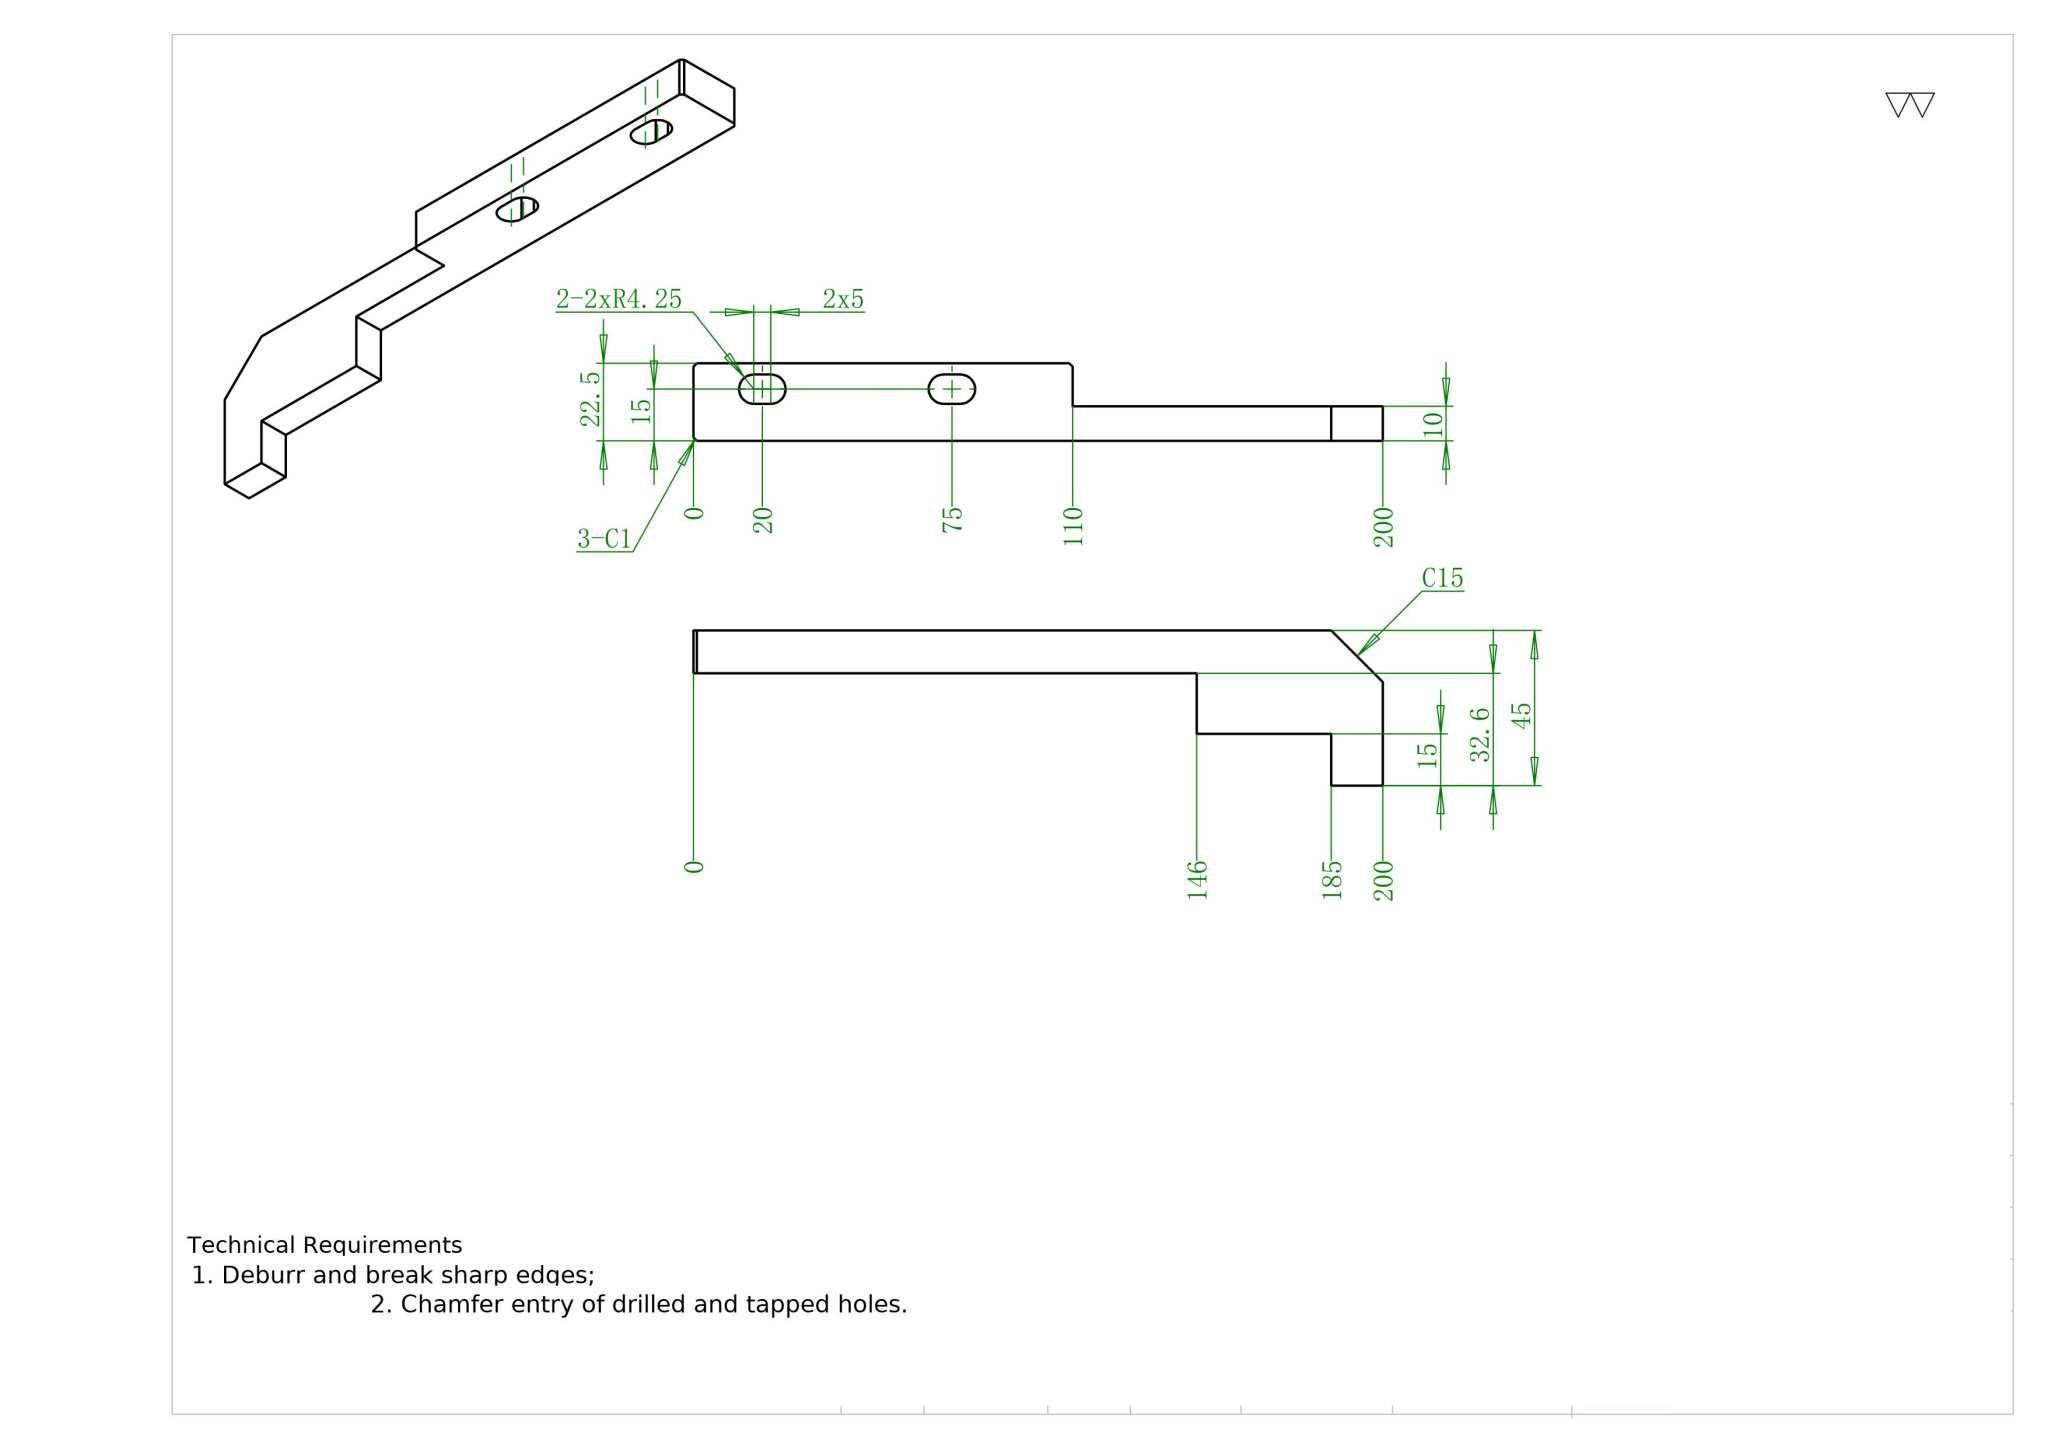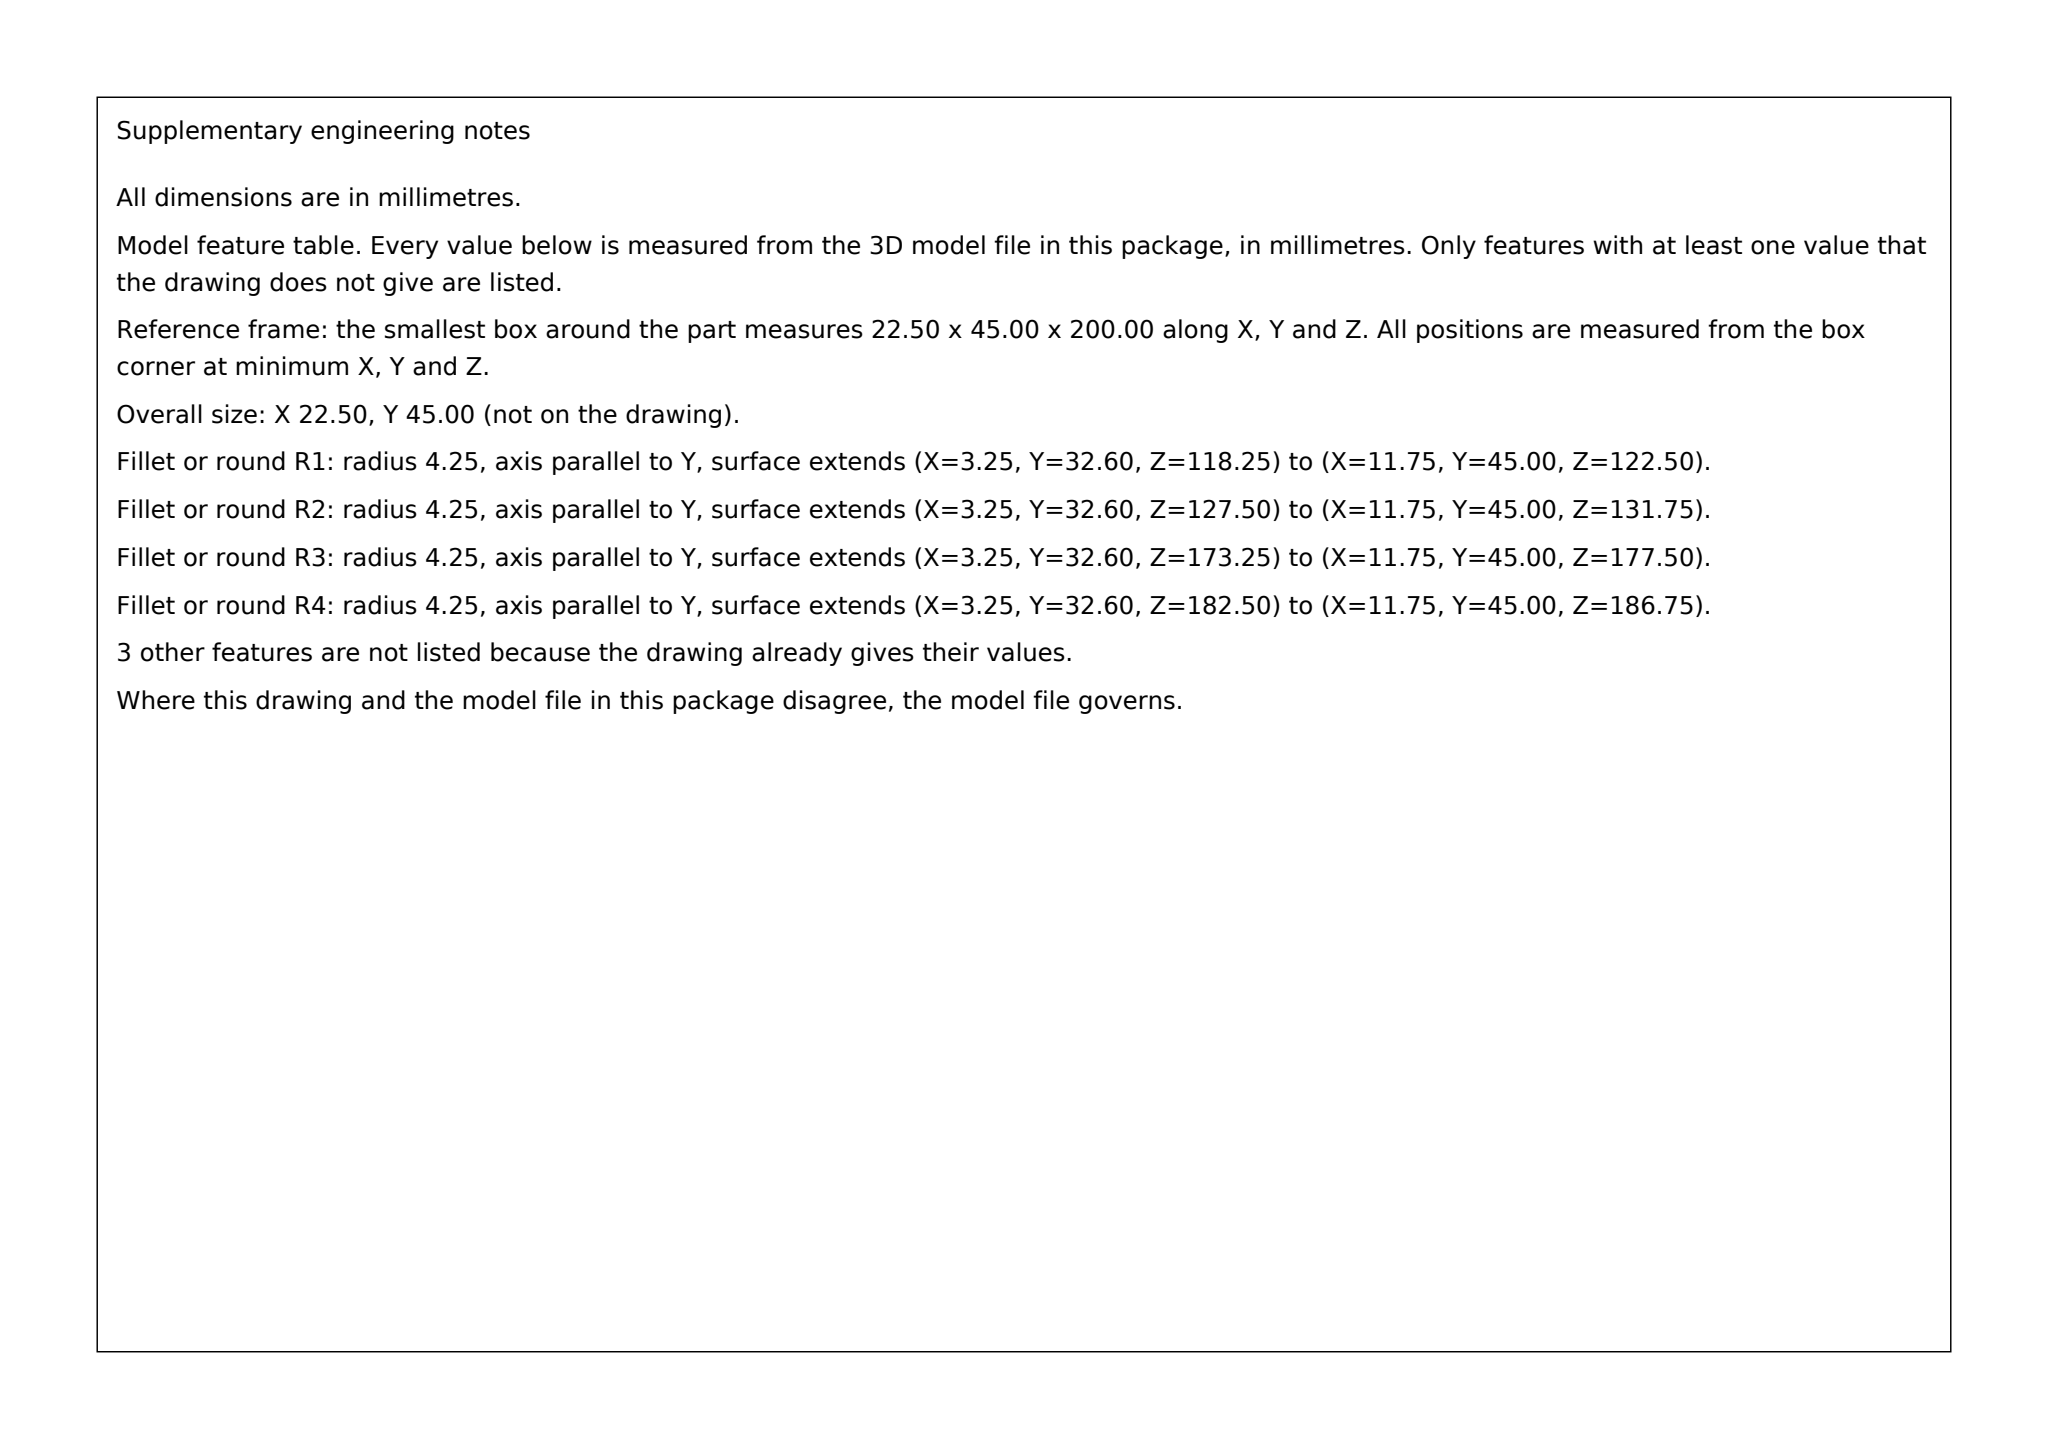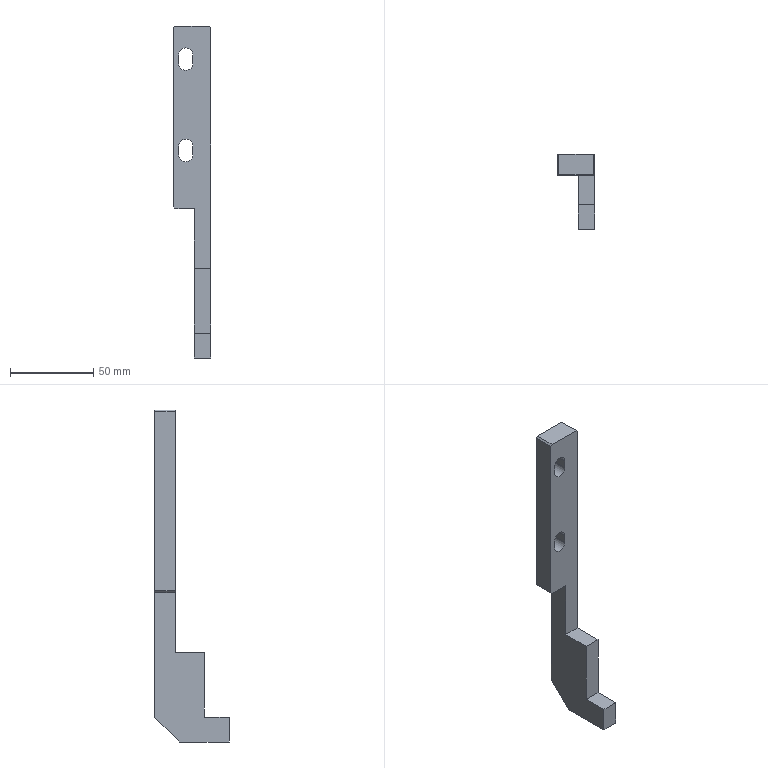Part | SolidWorks | mm | 1 solid | 26 faces | box 22.5 x 45 x 200 mm | volume 49999 mm3 | plane 20 | cylinder 6 | commonest cylinder face diameters 8.5 x6
build123d program:
from build123d import *

# Parameters (mm, degrees)
SKETCH1_W                  = 10
SKETCH1_H                  = 200
BOSS_EXTRUDE1_DEPTH        = 30
SKETCH2_W                  = 10
SKETCH2_H                  = 15
BOSS_EXTRUDE2_DEPTH        = 15
SKETCH3_W                  = 146
SKETCH3_H                  = 17.6
CUT_EXTRUDE1_DEPTH         = 105.881
SKETCH4_W                  = 110
SKETCH4_H                  = 12.4
BOSS_EXTRUDE3_DEPTH        = 12.5
CHAMFER1_SIZE              = 15
F_8_5_8_5_DIAMETER_HOLE1_D = 8.5
CUT_EXTRUDE2_DEPTH         = 112.046
CHAMFER2_SIZE              = 1


with BuildPart() as part:
    # Sketch1 → Boss-Extrude1 (new body)
    with BuildSketch(Plane(origin=(0, 0, 0), x_dir=(1, 0, 0), z_dir=(0, 1, 0))):
        Rectangle(SKETCH1_W, SKETCH1_H)
    extrude(amount=BOSS_EXTRUDE1_DEPTH)

    # Sketch2 → Boss-Extrude2 (add)
    with BuildSketch(Plane.XZ):
        with Locations((0, -92.5)):
            Rectangle(SKETCH2_W, SKETCH2_H)
    extrude(amount=BOSS_EXTRUDE2_DEPTH)

    # Sketch3 → Cut-Extrude1 (cut, through all)
    with BuildSketch(Plane.ZY.offset(5)):
        with Locations((27, 8.8)):
            Rectangle(SKETCH3_W, SKETCH3_H)
    extrude(amount=-CUT_EXTRUDE1_DEPTH, mode=Mode.SUBTRACT)

    # Sketch4 → Boss-Extrude3 (add)
    with BuildSketch(Plane.ZY.offset(5)):
        with Locations((45, 23.8)):
            Rectangle(SKETCH4_W, SKETCH4_H)
    extrude(amount=BOSS_EXTRUDE3_DEPTH)

    # Chamfer1
    chamfer1_edges = [part.edges().sort_by_distance(p)[0] for p in [
        (0, 30, -100),
    ]]
    chamfer(chamfer1_edges, length=CHAMFER1_SIZE)

    # 8.5 _8.5_ Diameter Hole1 (through all)
    with Locations(Plane(origin=(0, 30, 0), x_dir=(1, 0, 0), z_dir=(0, 1, 0))):
        with Locations((-10, -80), (-10, -25)):
            Hole(F_8_5_8_5_DIAMETER_HOLE1_D / 2)

    # Sketch7 → Cut-Extrude2 (cut, through all)
    with BuildSketch(Plane(origin=(0, 30, 0), x_dir=(1, 0, 0), z_dir=(0, 1, 0))):
        with BuildLine():
            Line((-14.25, -27.5), (-14.25, -22.5))
            ThreePointArc((-14.25, -22.5), (-10, -18.25), (-5.75, -22.5))
            Line((-5.75, -22.5), (-5.75, -27.5))
            ThreePointArc((-5.75, -27.5), (-10, -31.75), (-14.25, -27.5))
        make_face()
        with BuildLine():
            Line((-14.25, -82.5), (-14.25, -77.5))
            ThreePointArc((-14.25, -77.5), (-10, -73.25), (-5.75, -77.5))
            Line((-5.75, -77.5), (-5.75, -82.5))
            ThreePointArc((-5.75, -82.5), (-10, -86.75), (-14.25, -82.5))
        make_face()
    extrude(amount=-CUT_EXTRUDE2_DEPTH, mode=Mode.SUBTRACT)

    # Chamfer2
    chamfer2_edges = [part.edges().sort_by_distance(p)[0] for p in [
        (-17.5, 23.8, -10),
        (5, 23.8, 100),
        (-17.5, 23.8, 100),
    ]]
    chamfer(chamfer2_edges, length=CHAMFER2_SIZE)


solid = part.part
STEP:
#1=CARTESIAN_POINT('',(-10.,17.6,86.75));
#2=VERTEX_POINT('',#1);
#3=CARTESIAN_POINT('',(-5.75,17.6,82.5));
#4=VERTEX_POINT('',#3);
#5=CARTESIAN_POINT('',(-10.,17.6,82.5));
#6=DIRECTION('',(0.,1.,0.));
#7=DIRECTION('',(0.,0.,1.));
#8=AXIS2_PLACEMENT_3D('',#5,#6,#7);
#9=CIRCLE('',#8,4.25);
#10=EDGE_CURVE('',#2,#4,#9,.T.);
#11=ORIENTED_EDGE('',*,*,#10,.F.);
#12=CARTESIAN_POINT('',(-10.,30.,86.75));
#13=VERTEX_POINT('',#12);
#14=CARTESIAN_POINT('',(-10.,-15.,86.75));
#15=DIRECTION('',(0.,1.,0.));
#16=VECTOR('',#15,1000.);
#17=LINE('',#14,#16);
#18=EDGE_CURVE('',#2,#13,#17,.T.);
#19=ORIENTED_EDGE('',*,*,#18,.T.);
#20=CARTESIAN_POINT('',(-5.75,30.,82.5));
#21=VERTEX_POINT('',#20);
#22=CARTESIAN_POINT('',(-10.,30.,82.5));
#23=DIRECTION('',(0.,1.,0.));
#24=DIRECTION('',(0.,0.,1.));
#25=AXIS2_PLACEMENT_3D('',#22,#23,#24);
#26=CIRCLE('',#25,4.25);
#27=EDGE_CURVE('',#13,#21,#26,.T.);
#28=ORIENTED_EDGE('',*,*,#27,.T.);
#29=CARTESIAN_POINT('',(-5.75,-15.,82.5));
#30=DIRECTION('',(0.,1.,0.));
#31=VECTOR('',#30,1000.);
#32=LINE('',#29,#31);
#33=EDGE_CURVE('',#4,#21,#32,.T.);
#34=ORIENTED_EDGE('',*,*,#33,.F.);
#35=EDGE_LOOP('',(#11,#19,#28,#34));
#36=FACE_OUTER_BOUND('',#35,.T.);
#37=CARTESIAN_POINT('',(-10.,-15.,82.5));
#38=DIRECTION('',(0.,1.,0.));
#39=DIRECTION('',(0.,0.,1.));
#40=AXIS2_PLACEMENT_3D('',#37,#38,#39);
#41=CYLINDRICAL_SURFACE('',#40,4.25);
#42=ADVANCED_FACE('',(#36),#41,.F.);
#43=CARTESIAN_POINT('',(-10.,17.6,31.75));
#44=VERTEX_POINT('',#43);
#45=CARTESIAN_POINT('',(-5.75,17.6,27.5));
#46=VERTEX_POINT('',#45);
#47=CARTESIAN_POINT('',(-10.,17.6,27.5));
#48=DIRECTION('',(0.,1.,0.));
#49=DIRECTION('',(0.,0.,1.));
#50=AXIS2_PLACEMENT_3D('',#47,#48,#49);
#51=CIRCLE('',#50,4.25);
#52=EDGE_CURVE('',#44,#46,#51,.T.);
#53=ORIENTED_EDGE('',*,*,#52,.F.);
#54=CARTESIAN_POINT('',(-10.,30.,31.75));
#55=VERTEX_POINT('',#54);
#56=CARTESIAN_POINT('',(-10.,-15.,31.75));
#57=DIRECTION('',(0.,1.,0.));
#58=VECTOR('',#57,1000.);
#59=LINE('',#56,#58);
#60=EDGE_CURVE('',#44,#55,#59,.T.);
#61=ORIENTED_EDGE('',*,*,#60,.T.);
#62=CARTESIAN_POINT('',(-5.75,30.,27.5));
#63=VERTEX_POINT('',#62);
#64=CARTESIAN_POINT('',(-10.,30.,27.5));
#65=DIRECTION('',(0.,1.,0.));
#66=DIRECTION('',(0.,0.,1.));
#67=AXIS2_PLACEMENT_3D('',#64,#65,#66);
#68=CIRCLE('',#67,4.25);
#69=EDGE_CURVE('',#55,#63,#68,.T.);
#70=ORIENTED_EDGE('',*,*,#69,.T.);
#71=CARTESIAN_POINT('',(-5.75,-15.,27.5));
#72=DIRECTION('',(0.,1.,0.));
#73=VECTOR('',#72,1000.);
#74=LINE('',#71,#73);
#75=EDGE_CURVE('',#46,#63,#74,.T.);
#76=ORIENTED_EDGE('',*,*,#75,.F.);
#77=EDGE_LOOP('',(#53,#61,#70,#76));
#78=FACE_OUTER_BOUND('',#77,.T.);
#79=CARTESIAN_POINT('',(-10.,-15.,27.5));
#80=DIRECTION('',(0.,1.,0.));
#81=DIRECTION('',(0.,0.,1.));
#82=AXIS2_PLACEMENT_3D('',#79,#80,#81);
#83=CYLINDRICAL_SURFACE('',#82,4.25);
#84=ADVANCED_FACE('',(#78),#83,.F.);
#85=CARTESIAN_POINT('',(-5.,30.,-85.));
#86=VERTEX_POINT('',#85);
#87=CARTESIAN_POINT('',(-5.,30.,-10.));
#88=VERTEX_POINT('',#87);
#89=CARTESIAN_POINT('',(-5.,30.,-100.));
#90=DIRECTION('',(0.,0.,1.));
#91=VECTOR('',#90,1000.);
#92=LINE('',#89,#91);
#93=EDGE_CURVE('',#86,#88,#92,.T.);
#94=ORIENTED_EDGE('',*,*,#93,.F.);
#95=CARTESIAN_POINT('',(-5.,15.,-100.));
#96=VERTEX_POINT('',#95);
#97=CARTESIAN_POINT('',(-5.,30.,-85.));
#98=DIRECTION('',(-0.,-0.7071,-0.7071));
#99=VECTOR('',#98,1000.);
#100=LINE('',#97,#99);
#101=EDGE_CURVE('',#86,#96,#100,.T.);
#102=ORIENTED_EDGE('',*,*,#101,.T.);
#103=CARTESIAN_POINT('',(-5.,-15.,-100.));
#104=VERTEX_POINT('',#103);
#105=CARTESIAN_POINT('',(-5.,30.,-100.));
#106=DIRECTION('',(0.,-1.,0.));
#107=VECTOR('',#106,1000.);
#108=LINE('',#105,#107);
#109=EDGE_CURVE('',#96,#104,#108,.T.);
#110=ORIENTED_EDGE('',*,*,#109,.T.);
#111=CARTESIAN_POINT('',(-5.,-15.,-85.));
#112=VERTEX_POINT('',#111);
#113=CARTESIAN_POINT('',(-5.,-15.,-100.));
#114=DIRECTION('',(0.,0.,-1.));
#115=VECTOR('',#114,1000.);
#116=LINE('',#113,#115);
#117=EDGE_CURVE('',#112,#104,#116,.T.);
#118=ORIENTED_EDGE('',*,*,#117,.F.);
#119=CARTESIAN_POINT('',(-5.,0.,-85.));
#120=VERTEX_POINT('',#119);
#121=CARTESIAN_POINT('',(-5.,-15.,-85.));
#122=DIRECTION('',(0.,1.,0.));
#123=VECTOR('',#122,1000.);
#124=LINE('',#121,#123);
#125=EDGE_CURVE('',#112,#120,#124,.T.);
#126=ORIENTED_EDGE('',*,*,#125,.T.);
#127=CARTESIAN_POINT('',(-5.,0.,-46.));
#128=VERTEX_POINT('',#127);
#129=CARTESIAN_POINT('',(-5.,0.,-100.));
#130=DIRECTION('',(0.,0.,1.));
#131=VECTOR('',#130,1000.);
#132=LINE('',#129,#131);
#133=EDGE_CURVE('',#120,#128,#132,.T.);
#134=ORIENTED_EDGE('',*,*,#133,.T.);
#135=CARTESIAN_POINT('',(-5.,17.6,-46.));
#136=VERTEX_POINT('',#135);
#137=CARTESIAN_POINT('',(-5.,0.,-46.));
#138=DIRECTION('',(0.,-1.,0.));
#139=VECTOR('',#138,1000.);
#140=LINE('',#137,#139);
#141=EDGE_CURVE('',#136,#128,#140,.T.);
#142=ORIENTED_EDGE('',*,*,#141,.F.);
#143=CARTESIAN_POINT('',(-5.,17.6,-10.));
#144=VERTEX_POINT('',#143);
#145=CARTESIAN_POINT('',(-5.,17.6,-46.));
#146=DIRECTION('',(-0.,0.,-1.));
#147=VECTOR('',#146,1000.);
#148=LINE('',#145,#147);
#149=EDGE_CURVE('',#144,#136,#148,.T.);
#150=ORIENTED_EDGE('',*,*,#149,.F.);
#151=CARTESIAN_POINT('',(-5.,30.,-10.));
#152=DIRECTION('',(0.,-1.,0.));
#153=VECTOR('',#152,1000.);
#154=LINE('',#151,#153);
#155=EDGE_CURVE('',#88,#144,#154,.T.);
#156=ORIENTED_EDGE('',*,*,#155,.F.);
#157=EDGE_LOOP('',(#94,#102,#110,#118,#126,#134,#142,#150,#156));
#158=FACE_OUTER_BOUND('',#157,.T.);
#159=CARTESIAN_POINT('',(-5.,30.,-100.));
#160=DIRECTION('',(1.,0.,-0.));
#161=DIRECTION('',(-0.,0.,-1.));
#162=AXIS2_PLACEMENT_3D('',#159,#160,#161);
#163=PLANE('',#162);
#164=ADVANCED_FACE('',(#158),#163,.F.);
#165=CARTESIAN_POINT('',(5.,0.,-46.));
#166=VERTEX_POINT('',#165);
#167=CARTESIAN_POINT('',(5.,0.,-85.));
#168=VERTEX_POINT('',#167);
#169=CARTESIAN_POINT('',(5.,0.,-100.));
#170=DIRECTION('',(-0.,0.,-1.));
#171=VECTOR('',#170,1000.);
#172=LINE('',#169,#171);
#173=EDGE_CURVE('',#166,#168,#172,.T.);
#174=ORIENTED_EDGE('',*,*,#173,.F.);
#175=CARTESIAN_POINT('',(5.,0.,-46.));
#176=DIRECTION('',(-1.,0.,0.));
#177=VECTOR('',#176,1000.);
#178=LINE('',#175,#177);
#179=EDGE_CURVE('',#166,#128,#178,.T.);
#180=ORIENTED_EDGE('',*,*,#179,.T.);
#181=ORIENTED_EDGE('',*,*,#133,.F.);
#182=CARTESIAN_POINT('',(5.,0.,-85.));
#183=DIRECTION('',(-1.,0.,0.));
#184=VECTOR('',#183,1000.);
#185=LINE('',#182,#184);
#186=EDGE_CURVE('',#168,#120,#185,.T.);
#187=ORIENTED_EDGE('',*,*,#186,.F.);
#188=EDGE_LOOP('',(#174,#180,#181,#187));
#189=FACE_OUTER_BOUND('',#188,.T.);
#190=CARTESIAN_POINT('',(0.,0.,0.));
#191=DIRECTION('',(0.,1.,0.));
#192=DIRECTION('',(0.,0.,1.));
#193=AXIS2_PLACEMENT_3D('',#190,#191,#192);
#194=PLANE('',#193);
#195=ADVANCED_FACE('',(#189),#194,.F.);
#196=CARTESIAN_POINT('',(5.,30.,99.));
#197=VERTEX_POINT('',#196);
#198=CARTESIAN_POINT('',(5.,30.,-85.));
#199=VERTEX_POINT('',#198);
#200=CARTESIAN_POINT('',(5.,30.,-100.));
#201=DIRECTION('',(-0.,0.,-1.));
#202=VECTOR('',#201,1000.);
#203=LINE('',#200,#202);
#204=EDGE_CURVE('',#197,#199,#203,.T.);
#205=ORIENTED_EDGE('',*,*,#204,.F.);
#206=CARTESIAN_POINT('',(5.,17.6,99.));
#207=VERTEX_POINT('',#206);
#208=CARTESIAN_POINT('',(5.,30.,99.));
#209=DIRECTION('',(0.,-1.,0.));
#210=VECTOR('',#209,1000.);
#211=LINE('',#208,#210);
#212=EDGE_CURVE('',#197,#207,#211,.T.);
#213=ORIENTED_EDGE('',*,*,#212,.T.);
#214=CARTESIAN_POINT('',(5.,17.6,-46.));
#215=VERTEX_POINT('',#214);
#216=CARTESIAN_POINT('',(5.,17.6,-100.));
#217=DIRECTION('',(-0.,0.,-1.));
#218=VECTOR('',#217,1000.);
#219=LINE('',#216,#218);
#220=EDGE_CURVE('',#207,#215,#219,.T.);
#221=ORIENTED_EDGE('',*,*,#220,.T.);
#222=CARTESIAN_POINT('',(5.,30.,-46.));
#223=DIRECTION('',(0.,-1.,0.));
#224=VECTOR('',#223,1000.);
#225=LINE('',#222,#224);
#226=EDGE_CURVE('',#215,#166,#225,.T.);
#227=ORIENTED_EDGE('',*,*,#226,.T.);
#228=ORIENTED_EDGE('',*,*,#173,.T.);
#229=CARTESIAN_POINT('',(5.,-15.,-85.));
#230=VERTEX_POINT('',#229);
#231=CARTESIAN_POINT('',(5.,-15.,-85.));
#232=DIRECTION('',(0.,1.,0.));
#233=VECTOR('',#232,1000.);
#234=LINE('',#231,#233);
#235=EDGE_CURVE('',#230,#168,#234,.T.);
#236=ORIENTED_EDGE('',*,*,#235,.F.);
#237=CARTESIAN_POINT('',(5.,-15.,-100.));
#238=VERTEX_POINT('',#237);
#239=CARTESIAN_POINT('',(5.,-15.,-100.));
#240=DIRECTION('',(0.,0.,1.));
#241=VECTOR('',#240,1000.);
#242=LINE('',#239,#241);
#243=EDGE_CURVE('',#238,#230,#242,.T.);
#244=ORIENTED_EDGE('',*,*,#243,.F.);
#245=CARTESIAN_POINT('',(5.,15.,-100.));
#246=VERTEX_POINT('',#245);
#247=CARTESIAN_POINT('',(5.,30.,-100.));
#248=DIRECTION('',(0.,-1.,0.));
#249=VECTOR('',#248,1000.);
#250=LINE('',#247,#249);
#251=EDGE_CURVE('',#246,#238,#250,.T.);
#252=ORIENTED_EDGE('',*,*,#251,.F.);
#253=CARTESIAN_POINT('',(5.,30.,-85.));
#254=DIRECTION('',(0.,0.7071,0.7071));
#255=VECTOR('',#254,1000.);
#256=LINE('',#253,#255);
#257=EDGE_CURVE('',#246,#199,#256,.T.);
#258=ORIENTED_EDGE('',*,*,#257,.T.);
#259=EDGE_LOOP('',(#205,#213,#221,#227,#228,#236,#244,#252,#258));
#260=FACE_OUTER_BOUND('',#259,.T.);
#261=CARTESIAN_POINT('',(5.,30.,-100.));
#262=DIRECTION('',(-1.,0.,0.));
#263=DIRECTION('',(0.,0.,1.));
#264=AXIS2_PLACEMENT_3D('',#261,#262,#263);
#265=PLANE('',#264);
#266=ADVANCED_FACE('',(#260),#265,.F.);
#267=ORIENTED_EDGE('',*,*,#109,.F.);
#268=CARTESIAN_POINT('',(5.,15.,-100.));
#269=DIRECTION('',(1.,0.,0.));
#270=VECTOR('',#269,1000.);
#271=LINE('',#268,#270);
#272=EDGE_CURVE('',#96,#246,#271,.T.);
#273=ORIENTED_EDGE('',*,*,#272,.T.);
#274=ORIENTED_EDGE('',*,*,#251,.T.);
#275=CARTESIAN_POINT('',(5.,-15.,-100.));
#276=DIRECTION('',(1.,0.,0.));
#277=VECTOR('',#276,1000.);
#278=LINE('',#275,#277);
#279=EDGE_CURVE('',#104,#238,#278,.T.);
#280=ORIENTED_EDGE('',*,*,#279,.F.);
#281=EDGE_LOOP('',(#267,#273,#274,#280));
#282=FACE_OUTER_BOUND('',#281,.T.);
#283=CARTESIAN_POINT('',(-5.,30.,-100.));
#284=DIRECTION('',(0.,0.,1.));
#285=DIRECTION('',(1.,0.,0.));
#286=AXIS2_PLACEMENT_3D('',#283,#284,#285);
#287=PLANE('',#286);
#288=ADVANCED_FACE('',(#282),#287,.F.);
#289=CARTESIAN_POINT('',(-16.5,17.6,100.));
#290=VERTEX_POINT('',#289);
#291=CARTESIAN_POINT('',(4.,17.6,100.));
#292=VERTEX_POINT('',#291);
#293=CARTESIAN_POINT('',(-5.,17.6,100.));
#294=DIRECTION('',(1.,0.,0.));
#295=VECTOR('',#294,1000.);
#296=LINE('',#293,#295);
#297=EDGE_CURVE('',#290,#292,#296,.T.);
#298=ORIENTED_EDGE('',*,*,#297,.T.);
#299=CARTESIAN_POINT('',(4.,30.,100.));
#300=VERTEX_POINT('',#299);
#301=CARTESIAN_POINT('',(4.,30.,100.));
#302=DIRECTION('',(0.,1.,0.));
#303=VECTOR('',#302,1000.);
#304=LINE('',#301,#303);
#305=EDGE_CURVE('',#292,#300,#304,.T.);
#306=ORIENTED_EDGE('',*,*,#305,.T.);
#307=CARTESIAN_POINT('',(-16.5,30.,100.));
#308=VERTEX_POINT('',#307);
#309=CARTESIAN_POINT('',(-5.,30.,100.));
#310=DIRECTION('',(1.,0.,0.));
#311=VECTOR('',#310,1000.);
#312=LINE('',#309,#311);
#313=EDGE_CURVE('',#308,#300,#312,.T.);
#314=ORIENTED_EDGE('',*,*,#313,.F.);
#315=CARTESIAN_POINT('',(-16.5,30.,100.));
#316=DIRECTION('',(0.,-1.,0.));
#317=VECTOR('',#316,1000.);
#318=LINE('',#315,#317);
#319=EDGE_CURVE('',#308,#290,#318,.T.);
#320=ORIENTED_EDGE('',*,*,#319,.T.);
#321=EDGE_LOOP('',(#298,#306,#314,#320));
#322=FACE_OUTER_BOUND('',#321,.T.);
#323=CARTESIAN_POINT('',(-5.,30.,100.));
#324=DIRECTION('',(0.,0.,-1.));
#325=DIRECTION('',(-1.,0.,0.));
#326=AXIS2_PLACEMENT_3D('',#323,#324,#325);
#327=PLANE('',#326);
#328=ADVANCED_FACE('',(#322),#327,.F.);
#329=CARTESIAN_POINT('',(-14.25,30.,82.5));
#330=VERTEX_POINT('',#329);
#331=CARTESIAN_POINT('',(-10.,30.,82.5));
#332=DIRECTION('',(0.,1.,0.));
#333=DIRECTION('',(0.,0.,1.));
#334=AXIS2_PLACEMENT_3D('',#331,#332,#333);
#335=CIRCLE('',#334,4.25);
#336=EDGE_CURVE('',#330,#13,#335,.T.);
#337=ORIENTED_EDGE('',*,*,#336,.F.);
#338=CARTESIAN_POINT('',(-14.25,30.,77.5));
#339=VERTEX_POINT('',#338);
#340=CARTESIAN_POINT('',(-14.25,30.,82.5));
#341=DIRECTION('',(0.,0.,1.));
#342=VECTOR('',#341,1000.);
#343=LINE('',#340,#342);
#344=EDGE_CURVE('',#339,#330,#343,.T.);
#345=ORIENTED_EDGE('',*,*,#344,.F.);
#346=CARTESIAN_POINT('',(-5.75,30.,77.5));
#347=VERTEX_POINT('',#346);
#348=CARTESIAN_POINT('',(-10.,30.,77.5));
#349=DIRECTION('',(0.,1.,0.));
#350=DIRECTION('',(0.,0.,1.));
#351=AXIS2_PLACEMENT_3D('',#348,#349,#350);
#352=CIRCLE('',#351,4.25);
#353=EDGE_CURVE('',#347,#339,#352,.T.);
#354=ORIENTED_EDGE('',*,*,#353,.F.);
#355=CARTESIAN_POINT('',(-5.75,30.,82.5));
#356=DIRECTION('',(0.,0.,-1.));
#357=VECTOR('',#356,1000.);
#358=LINE('',#355,#357);
#359=EDGE_CURVE('',#21,#347,#358,.T.);
#360=ORIENTED_EDGE('',*,*,#359,.F.);
#361=ORIENTED_EDGE('',*,*,#27,.F.);
#362=EDGE_LOOP('',(#337,#345,#354,#360,#361));
#363=FACE_BOUND('',#362,.T.);
#364=CARTESIAN_POINT('',(-14.25,30.,27.5));
#365=VERTEX_POINT('',#364);
#366=CARTESIAN_POINT('',(-10.,30.,27.5));
#367=DIRECTION('',(0.,1.,0.));
#368=DIRECTION('',(0.,0.,1.));
#369=AXIS2_PLACEMENT_3D('',#366,#367,#368);
#370=CIRCLE('',#369,4.25);
#371=EDGE_CURVE('',#365,#55,#370,.T.);
#372=ORIENTED_EDGE('',*,*,#371,.F.);
#373=CARTESIAN_POINT('',(-14.25,30.,22.5));
#374=VERTEX_POINT('',#373);
#375=CARTESIAN_POINT('',(-14.25,30.,27.5));
#376=DIRECTION('',(0.,0.,1.));
#377=VECTOR('',#376,1000.);
#378=LINE('',#375,#377);
#379=EDGE_CURVE('',#374,#365,#378,.T.);
#380=ORIENTED_EDGE('',*,*,#379,.F.);
#381=CARTESIAN_POINT('',(-5.75,30.,22.5));
#382=VERTEX_POINT('',#381);
#383=CARTESIAN_POINT('',(-10.,30.,22.5));
#384=DIRECTION('',(0.,1.,0.));
#385=DIRECTION('',(0.,0.,1.));
#386=AXIS2_PLACEMENT_3D('',#383,#384,#385);
#387=CIRCLE('',#386,4.25);
#388=EDGE_CURVE('',#382,#374,#387,.T.);
#389=ORIENTED_EDGE('',*,*,#388,.F.);
#390=CARTESIAN_POINT('',(-5.75,30.,27.5));
#391=DIRECTION('',(-0.,0.,-1.));
#392=VECTOR('',#391,1000.);
#393=LINE('',#390,#392);
#394=EDGE_CURVE('',#63,#382,#393,.T.);
#395=ORIENTED_EDGE('',*,*,#394,.F.);
#396=ORIENTED_EDGE('',*,*,#69,.F.);
#397=EDGE_LOOP('',(#372,#380,#389,#395,#396));
#398=FACE_BOUND('',#397,.T.);
#399=CARTESIAN_POINT('',(-16.5,30.,-10.));
#400=VERTEX_POINT('',#399);
#401=CARTESIAN_POINT('',(-17.5,30.,-10.));
#402=DIRECTION('',(1.,0.,-0.));
#403=VECTOR('',#402,1000.);
#404=LINE('',#401,#403);
#405=EDGE_CURVE('',#400,#88,#404,.T.);
#406=ORIENTED_EDGE('',*,*,#405,.F.);
#407=CARTESIAN_POINT('',(-17.5,30.,-9.));
#408=VERTEX_POINT('',#407);
#409=CARTESIAN_POINT('',(-13.25,30.,-13.25));
#410=DIRECTION('',(-0.7071,0.,0.7071));
#411=VECTOR('',#410,1000.);
#412=LINE('',#409,#411);
#413=EDGE_CURVE('',#400,#408,#412,.T.);
#414=ORIENTED_EDGE('',*,*,#413,.T.);
#415=CARTESIAN_POINT('',(-17.5,30.,99.));
#416=VERTEX_POINT('',#415);
#417=CARTESIAN_POINT('',(-17.5,30.,100.));
#418=DIRECTION('',(-0.,-0.,-1.));
#419=VECTOR('',#418,1000.);
#420=LINE('',#417,#419);
#421=EDGE_CURVE('',#416,#408,#420,.T.);
#422=ORIENTED_EDGE('',*,*,#421,.F.);
#423=CARTESIAN_POINT('',(-58.25,30.,58.25));
#424=DIRECTION('',(0.7071,0.,0.7071));
#425=VECTOR('',#424,1000.);
#426=LINE('',#423,#425);
#427=EDGE_CURVE('',#416,#308,#426,.T.);
#428=ORIENTED_EDGE('',*,*,#427,.T.);
#429=ORIENTED_EDGE('',*,*,#313,.T.);
#430=CARTESIAN_POINT('',(52.,30.,52.));
#431=DIRECTION('',(0.7071,0.,-0.7071));
#432=VECTOR('',#431,1000.);
#433=LINE('',#430,#432);
#434=EDGE_CURVE('',#300,#197,#433,.T.);
#435=ORIENTED_EDGE('',*,*,#434,.T.);
#436=ORIENTED_EDGE('',*,*,#204,.T.);
#437=CARTESIAN_POINT('',(-5.,30.,-85.));
#438=DIRECTION('',(-1.,0.,0.));
#439=VECTOR('',#438,1000.);
#440=LINE('',#437,#439);
#441=EDGE_CURVE('',#199,#86,#440,.T.);
#442=ORIENTED_EDGE('',*,*,#441,.T.);
#443=ORIENTED_EDGE('',*,*,#93,.T.);
#444=EDGE_LOOP('',(#406,#414,#422,#428,#429,#435,#436,#442,#443));
#445=FACE_OUTER_BOUND('',#444,.T.);
#446=CARTESIAN_POINT('',(0.,30.,0.));
#447=DIRECTION('',(0.,1.,0.));
#448=DIRECTION('',(0.,0.,1.));
#449=AXIS2_PLACEMENT_3D('',#446,#447,#448);
#450=PLANE('',#449);
#451=ADVANCED_FACE('',(#363,#398,#445),#450,.T.);
#452=ORIENTED_EDGE('',*,*,#186,.T.);
#453=ORIENTED_EDGE('',*,*,#125,.F.);
#454=CARTESIAN_POINT('',(5.,-15.,-85.));
#455=DIRECTION('',(-1.,0.,0.));
#456=VECTOR('',#455,1000.);
#457=LINE('',#454,#456);
#458=EDGE_CURVE('',#230,#112,#457,.T.);
#459=ORIENTED_EDGE('',*,*,#458,.F.);
#460=ORIENTED_EDGE('',*,*,#235,.T.);
#461=EDGE_LOOP('',(#452,#453,#459,#460));
#462=FACE_OUTER_BOUND('',#461,.T.);
#463=CARTESIAN_POINT('',(5.,-15.,-85.));
#464=DIRECTION('',(0.,0.,-1.));
#465=DIRECTION('',(-1.,0.,0.));
#466=AXIS2_PLACEMENT_3D('',#463,#464,#465);
#467=PLANE('',#466);
#468=ADVANCED_FACE('',(#462),#467,.F.);
#469=ORIENTED_EDGE('',*,*,#243,.T.);
#470=ORIENTED_EDGE('',*,*,#458,.T.);
#471=ORIENTED_EDGE('',*,*,#117,.T.);
#472=ORIENTED_EDGE('',*,*,#279,.T.);
#473=EDGE_LOOP('',(#469,#470,#471,#472));
#474=FACE_OUTER_BOUND('',#473,.T.);
#475=CARTESIAN_POINT('',(0.,-15.,0.));
#476=DIRECTION('',(0.,-1.,0.));
#477=DIRECTION('',(0.,0.,-1.));
#478=AXIS2_PLACEMENT_3D('',#475,#476,#477);
#479=PLANE('',#478);
#480=ADVANCED_FACE('',(#474),#479,.T.);
#481=CARTESIAN_POINT('',(5.,17.6,-46.));
#482=DIRECTION('',(-1.,0.,0.));
#483=VECTOR('',#482,1000.);
#484=LINE('',#481,#483);
#485=EDGE_CURVE('',#215,#136,#484,.T.);
#486=ORIENTED_EDGE('',*,*,#485,.T.);
#487=ORIENTED_EDGE('',*,*,#141,.T.);
#488=ORIENTED_EDGE('',*,*,#179,.F.);
#489=ORIENTED_EDGE('',*,*,#226,.F.);
#490=EDGE_LOOP('',(#486,#487,#488,#489));
#491=FACE_OUTER_BOUND('',#490,.T.);
#492=CARTESIAN_POINT('',(5.,0.,-46.));
#493=DIRECTION('',(-0.,0.,-1.));
#494=DIRECTION('',(-1.,0.,0.));
#495=AXIS2_PLACEMENT_3D('',#492,#493,#494);
#496=PLANE('',#495);
#497=ADVANCED_FACE('',(#491),#496,.F.);
#498=CARTESIAN_POINT('',(-14.25,17.6,77.5));
#499=VERTEX_POINT('',#498);
#500=CARTESIAN_POINT('',(-14.25,17.6,82.5));
#501=VERTEX_POINT('',#500);
#502=CARTESIAN_POINT('',(-14.25,17.6,-46.));
#503=DIRECTION('',(0.,0.,1.));
#504=VECTOR('',#503,1000.);
#505=LINE('',#502,#504);
#506=EDGE_CURVE('',#499,#501,#505,.T.);
#507=ORIENTED_EDGE('',*,*,#506,.T.);
#508=CARTESIAN_POINT('',(-10.,17.6,82.5));
#509=DIRECTION('',(0.,1.,0.));
#510=DIRECTION('',(0.,0.,1.));
#511=AXIS2_PLACEMENT_3D('',#508,#509,#510);
#512=CIRCLE('',#511,4.25);
#513=EDGE_CURVE('',#501,#2,#512,.T.);
#514=ORIENTED_EDGE('',*,*,#513,.T.);
#515=ORIENTED_EDGE('',*,*,#10,.T.);
#516=CARTESIAN_POINT('',(-5.75,17.6,77.5));
#517=VERTEX_POINT('',#516);
#518=CARTESIAN_POINT('',(-5.75,17.6,-46.));
#519=DIRECTION('',(0.,0.,-1.));
#520=VECTOR('',#519,1000.);
#521=LINE('',#518,#520);
#522=EDGE_CURVE('',#4,#517,#521,.T.);
#523=ORIENTED_EDGE('',*,*,#522,.T.);
#524=CARTESIAN_POINT('',(-10.,17.6,77.5));
#525=DIRECTION('',(0.,1.,0.));
#526=DIRECTION('',(0.,0.,1.));
#527=AXIS2_PLACEMENT_3D('',#524,#525,#526);
#528=CIRCLE('',#527,4.25);
#529=EDGE_CURVE('',#517,#499,#528,.T.);
#530=ORIENTED_EDGE('',*,*,#529,.T.);
#531=EDGE_LOOP('',(#507,#514,#515,#523,#530));
#532=FACE_BOUND('',#531,.T.);
#533=CARTESIAN_POINT('',(-14.25,17.6,22.5));
#534=VERTEX_POINT('',#533);
#535=CARTESIAN_POINT('',(-14.25,17.6,27.5));
#536=VERTEX_POINT('',#535);
#537=CARTESIAN_POINT('',(-14.25,17.6,-46.));
#538=DIRECTION('',(0.,0.,1.));
#539=VECTOR('',#538,1000.);
#540=LINE('',#537,#539);
#541=EDGE_CURVE('',#534,#536,#540,.T.);
#542=ORIENTED_EDGE('',*,*,#541,.T.);
#543=CARTESIAN_POINT('',(-10.,17.6,27.5));
#544=DIRECTION('',(0.,1.,0.));
#545=DIRECTION('',(0.,0.,1.));
#546=AXIS2_PLACEMENT_3D('',#543,#544,#545);
#547=CIRCLE('',#546,4.25);
#548=EDGE_CURVE('',#536,#44,#547,.T.);
#549=ORIENTED_EDGE('',*,*,#548,.T.);
#550=ORIENTED_EDGE('',*,*,#52,.T.);
#551=CARTESIAN_POINT('',(-5.75,17.6,22.5));
#552=VERTEX_POINT('',#551);
#553=CARTESIAN_POINT('',(-5.75,17.6,-46.));
#554=DIRECTION('',(-0.,0.,-1.));
#555=VECTOR('',#554,1000.);
#556=LINE('',#553,#555);
#557=EDGE_CURVE('',#46,#552,#556,.T.);
#558=ORIENTED_EDGE('',*,*,#557,.T.);
#559=CARTESIAN_POINT('',(-10.,17.6,22.5));
#560=DIRECTION('',(0.,1.,0.));
#561=DIRECTION('',(0.,0.,1.));
#562=AXIS2_PLACEMENT_3D('',#559,#560,#561);
#563=CIRCLE('',#562,4.25);
#564=EDGE_CURVE('',#552,#534,#563,.T.);
#565=ORIENTED_EDGE('',*,*,#564,.T.);
#566=EDGE_LOOP('',(#542,#549,#550,#558,#565));
#567=FACE_BOUND('',#566,.T.);
#568=CARTESIAN_POINT('',(-17.5,17.6,-9.));
#569=VERTEX_POINT('',#568);
#570=CARTESIAN_POINT('',(-17.5,17.6,99.));
#571=VERTEX_POINT('',#570);
#572=CARTESIAN_POINT('',(-17.5,17.6,100.));
#573=DIRECTION('',(0.,-0.,1.));
#574=VECTOR('',#573,1000.);
#575=LINE('',#572,#574);
#576=EDGE_CURVE('',#569,#571,#575,.T.);
#577=ORIENTED_EDGE('',*,*,#576,.F.);
#578=CARTESIAN_POINT('',(-16.5,17.6,-10.));
#579=VERTEX_POINT('',#578);
#580=CARTESIAN_POINT('',(-17.5,17.6,-9.));
#581=DIRECTION('',(0.7071,0.,-0.7071));
#582=VECTOR('',#581,1000.);
#583=LINE('',#580,#582);
#584=EDGE_CURVE('',#569,#579,#583,.T.);
#585=ORIENTED_EDGE('',*,*,#584,.T.);
#586=CARTESIAN_POINT('',(-17.5,17.6,-10.));
#587=DIRECTION('',(1.,0.,-0.));
#588=VECTOR('',#587,1000.);
#589=LINE('',#586,#588);
#590=EDGE_CURVE('',#579,#144,#589,.T.);
#591=ORIENTED_EDGE('',*,*,#590,.T.);
#592=ORIENTED_EDGE('',*,*,#149,.T.);
#593=ORIENTED_EDGE('',*,*,#485,.F.);
#594=ORIENTED_EDGE('',*,*,#220,.F.);
#595=CARTESIAN_POINT('',(5.,17.6,99.));
#596=DIRECTION('',(-0.7071,0.,0.7071));
#597=VECTOR('',#596,1000.);
#598=LINE('',#595,#597);
#599=EDGE_CURVE('',#207,#292,#598,.T.);
#600=ORIENTED_EDGE('',*,*,#599,.T.);
#601=ORIENTED_EDGE('',*,*,#297,.F.);
#602=CARTESIAN_POINT('',(-17.5,17.6,99.));
#603=DIRECTION('',(-0.7071,0.,-0.7071));
#604=VECTOR('',#603,1000.);
#605=LINE('',#602,#604);
#606=EDGE_CURVE('',#290,#571,#605,.T.);
#607=ORIENTED_EDGE('',*,*,#606,.T.);
#608=EDGE_LOOP('',(#577,#585,#591,#592,#593,#594,#600,#601,#607));
#609=FACE_OUTER_BOUND('',#608,.T.);
#610=CARTESIAN_POINT('',(5.,17.6,-46.));
#611=DIRECTION('',(0.,1.,0.));
#612=DIRECTION('',(0.,0.,1.));
#613=AXIS2_PLACEMENT_3D('',#610,#611,#612);
#614=PLANE('',#613);
#615=ADVANCED_FACE('',(#532,#567,#609),#614,.F.);
#616=ORIENTED_EDGE('',*,*,#590,.F.);
#617=CARTESIAN_POINT('',(-16.5,30.,-10.));
#618=DIRECTION('',(0.,1.,0.));
#619=VECTOR('',#618,1000.);
#620=LINE('',#617,#619);
#621=EDGE_CURVE('',#579,#400,#620,.T.);
#622=ORIENTED_EDGE('',*,*,#621,.T.);
#623=ORIENTED_EDGE('',*,*,#405,.T.);
#624=ORIENTED_EDGE('',*,*,#155,.T.);
#625=EDGE_LOOP('',(#616,#622,#623,#624));
#626=FACE_OUTER_BOUND('',#625,.T.);
#627=CARTESIAN_POINT('',(-17.5,30.,-10.));
#628=DIRECTION('',(0.,0.,1.));
#629=DIRECTION('',(1.,0.,-0.));
#630=AXIS2_PLACEMENT_3D('',#627,#628,#629);
#631=PLANE('',#630);
#632=ADVANCED_FACE('',(#626),#631,.F.);
#633=ORIENTED_EDGE('',*,*,#421,.T.);
#634=CARTESIAN_POINT('',(-17.5,0.,-9.));
#635=DIRECTION('',(0.,-1.,0.));
#636=VECTOR('',#635,1000.);
#637=LINE('',#634,#636);
#638=EDGE_CURVE('',#408,#569,#637,.T.);
#639=ORIENTED_EDGE('',*,*,#638,.T.);
#640=ORIENTED_EDGE('',*,*,#576,.T.);
#641=CARTESIAN_POINT('',(-17.5,0.,99.));
#642=DIRECTION('',(0.,1.,0.));
#643=VECTOR('',#642,1000.);
#644=LINE('',#641,#643);
#645=EDGE_CURVE('',#571,#416,#644,.T.);
#646=ORIENTED_EDGE('',*,*,#645,.T.);
#647=EDGE_LOOP('',(#633,#639,#640,#646));
#648=FACE_OUTER_BOUND('',#647,.T.);
#649=CARTESIAN_POINT('',(-17.5,0.,0.));
#650=DIRECTION('',(1.,0.,-0.));
#651=DIRECTION('',(-0.,0.,-1.));
#652=AXIS2_PLACEMENT_3D('',#649,#650,#651);
#653=PLANE('',#652);
#654=ADVANCED_FACE('',(#648),#653,.F.);
#655=ORIENTED_EDGE('',*,*,#257,.F.);
#656=ORIENTED_EDGE('',*,*,#272,.F.);
#657=ORIENTED_EDGE('',*,*,#101,.F.);
#658=ORIENTED_EDGE('',*,*,#441,.F.);
#659=EDGE_LOOP('',(#655,#656,#657,#658));
#660=FACE_OUTER_BOUND('',#659,.T.);
#661=CARTESIAN_POINT('',(0.,30.,-85.));
#662=DIRECTION('',(0.,0.7071,-0.7071));
#663=DIRECTION('',(1.,0.,0.));
#664=AXIS2_PLACEMENT_3D('',#661,#662,#663);
#665=PLANE('',#664);
#666=ADVANCED_FACE('',(#660),#665,.T.);
#667=ORIENTED_EDGE('',*,*,#60,.F.);
#668=ORIENTED_EDGE('',*,*,#548,.F.);
#669=CARTESIAN_POINT('',(-14.25,-15.,27.5));
#670=DIRECTION('',(0.,1.,0.));
#671=VECTOR('',#670,1000.);
#672=LINE('',#669,#671);
#673=EDGE_CURVE('',#536,#365,#672,.T.);
#674=ORIENTED_EDGE('',*,*,#673,.T.);
#675=ORIENTED_EDGE('',*,*,#371,.T.);
#676=EDGE_LOOP('',(#667,#668,#674,#675));
#677=FACE_OUTER_BOUND('',#676,.T.);
#678=CARTESIAN_POINT('',(-10.,-15.,27.5));
#679=DIRECTION('',(0.,1.,0.));
#680=DIRECTION('',(0.,0.,1.));
#681=AXIS2_PLACEMENT_3D('',#678,#679,#680);
#682=CYLINDRICAL_SURFACE('',#681,4.25);
#683=ADVANCED_FACE('',(#677),#682,.F.);
#684=CARTESIAN_POINT('',(-5.75,-15.,22.5));
#685=DIRECTION('',(0.,1.,0.));
#686=VECTOR('',#685,1000.);
#687=LINE('',#684,#686);
#688=EDGE_CURVE('',#552,#382,#687,.T.);
#689=ORIENTED_EDGE('',*,*,#688,.T.);
#690=ORIENTED_EDGE('',*,*,#388,.T.);
#691=CARTESIAN_POINT('',(-14.25,-15.,22.5));
#692=DIRECTION('',(0.,1.,0.));
#693=VECTOR('',#692,1000.);
#694=LINE('',#691,#693);
#695=EDGE_CURVE('',#534,#374,#694,.T.);
#696=ORIENTED_EDGE('',*,*,#695,.F.);
#697=ORIENTED_EDGE('',*,*,#564,.F.);
#698=EDGE_LOOP('',(#689,#690,#696,#697));
#699=FACE_OUTER_BOUND('',#698,.T.);
#700=CARTESIAN_POINT('',(-10.,-15.,22.5));
#701=DIRECTION('',(0.,1.,0.));
#702=DIRECTION('',(0.,0.,1.));
#703=AXIS2_PLACEMENT_3D('',#700,#701,#702);
#704=CYLINDRICAL_SURFACE('',#703,4.25);
#705=ADVANCED_FACE('',(#699),#704,.F.);
#706=ORIENTED_EDGE('',*,*,#695,.T.);
#707=ORIENTED_EDGE('',*,*,#379,.T.);
#708=ORIENTED_EDGE('',*,*,#673,.F.);
#709=ORIENTED_EDGE('',*,*,#541,.F.);
#710=EDGE_LOOP('',(#706,#707,#708,#709));
#711=FACE_OUTER_BOUND('',#710,.T.);
#712=CARTESIAN_POINT('',(-14.25,-15.,27.5));
#713=DIRECTION('',(-1.,0.,0.));
#714=DIRECTION('',(0.,0.,1.));
#715=AXIS2_PLACEMENT_3D('',#712,#713,#714);
#716=PLANE('',#715);
#717=ADVANCED_FACE('',(#711),#716,.F.);
#718=ORIENTED_EDGE('',*,*,#75,.T.);
#719=ORIENTED_EDGE('',*,*,#394,.T.);
#720=ORIENTED_EDGE('',*,*,#688,.F.);
#721=ORIENTED_EDGE('',*,*,#557,.F.);
#722=EDGE_LOOP('',(#718,#719,#720,#721));
#723=FACE_OUTER_BOUND('',#722,.T.);
#724=CARTESIAN_POINT('',(-5.75,-15.,27.5));
#725=DIRECTION('',(1.,0.,-0.));
#726=DIRECTION('',(-0.,0.,-1.));
#727=AXIS2_PLACEMENT_3D('',#724,#725,#726);
#728=PLANE('',#727);
#729=ADVANCED_FACE('',(#723),#728,.F.);
#730=ORIENTED_EDGE('',*,*,#18,.F.);
#731=ORIENTED_EDGE('',*,*,#513,.F.);
#732=CARTESIAN_POINT('',(-14.25,-15.,82.5));
#733=DIRECTION('',(0.,1.,0.));
#734=VECTOR('',#733,1000.);
#735=LINE('',#732,#734);
#736=EDGE_CURVE('',#501,#330,#735,.T.);
#737=ORIENTED_EDGE('',*,*,#736,.T.);
#738=ORIENTED_EDGE('',*,*,#336,.T.);
#739=EDGE_LOOP('',(#730,#731,#737,#738));
#740=FACE_OUTER_BOUND('',#739,.T.);
#741=CARTESIAN_POINT('',(-10.,-15.,82.5));
#742=DIRECTION('',(0.,1.,0.));
#743=DIRECTION('',(0.,0.,1.));
#744=AXIS2_PLACEMENT_3D('',#741,#742,#743);
#745=CYLINDRICAL_SURFACE('',#744,4.25);
#746=ADVANCED_FACE('',(#740),#745,.F.);
#747=CARTESIAN_POINT('',(-5.75,-15.,77.5));
#748=DIRECTION('',(0.,1.,0.));
#749=VECTOR('',#748,1000.);
#750=LINE('',#747,#749);
#751=EDGE_CURVE('',#517,#347,#750,.T.);
#752=ORIENTED_EDGE('',*,*,#751,.T.);
#753=ORIENTED_EDGE('',*,*,#353,.T.);
#754=CARTESIAN_POINT('',(-14.25,-15.,77.5));
#755=DIRECTION('',(0.,1.,0.));
#756=VECTOR('',#755,1000.);
#757=LINE('',#754,#756);
#758=EDGE_CURVE('',#499,#339,#757,.T.);
#759=ORIENTED_EDGE('',*,*,#758,.F.);
#760=ORIENTED_EDGE('',*,*,#529,.F.);
#761=EDGE_LOOP('',(#752,#753,#759,#760));
#762=FACE_OUTER_BOUND('',#761,.T.);
#763=CARTESIAN_POINT('',(-10.,-15.,77.5));
#764=DIRECTION('',(0.,1.,0.));
#765=DIRECTION('',(0.,0.,1.));
#766=AXIS2_PLACEMENT_3D('',#763,#764,#765);
#767=CYLINDRICAL_SURFACE('',#766,4.25);
#768=ADVANCED_FACE('',(#762),#767,.F.);
#769=ORIENTED_EDGE('',*,*,#758,.T.);
#770=ORIENTED_EDGE('',*,*,#344,.T.);
#771=ORIENTED_EDGE('',*,*,#736,.F.);
#772=ORIENTED_EDGE('',*,*,#506,.F.);
#773=EDGE_LOOP('',(#769,#770,#771,#772));
#774=FACE_OUTER_BOUND('',#773,.T.);
#775=CARTESIAN_POINT('',(-14.25,-15.,82.5));
#776=DIRECTION('',(-1.,0.,0.));
#777=DIRECTION('',(0.,0.,1.));
#778=AXIS2_PLACEMENT_3D('',#775,#776,#777);
#779=PLANE('',#778);
#780=ADVANCED_FACE('',(#774),#779,.F.);
#781=ORIENTED_EDGE('',*,*,#33,.T.);
#782=ORIENTED_EDGE('',*,*,#359,.T.);
#783=ORIENTED_EDGE('',*,*,#751,.F.);
#784=ORIENTED_EDGE('',*,*,#522,.F.);
#785=EDGE_LOOP('',(#781,#782,#783,#784));
#786=FACE_OUTER_BOUND('',#785,.T.);
#787=CARTESIAN_POINT('',(-5.75,-15.,82.5));
#788=DIRECTION('',(1.,0.,0.));
#789=DIRECTION('',(0.,0.,-1.));
#790=AXIS2_PLACEMENT_3D('',#787,#788,#789);
#791=PLANE('',#790);
#792=ADVANCED_FACE('',(#786),#791,.F.);
#793=ORIENTED_EDGE('',*,*,#413,.F.);
#794=ORIENTED_EDGE('',*,*,#621,.F.);
#795=ORIENTED_EDGE('',*,*,#584,.F.);
#796=ORIENTED_EDGE('',*,*,#638,.F.);
#797=EDGE_LOOP('',(#793,#794,#795,#796));
#798=FACE_OUTER_BOUND('',#797,.T.);
#799=CARTESIAN_POINT('',(-17.5,0.,-9.));
#800=DIRECTION('',(0.7071,0.,0.7071));
#801=DIRECTION('',(0.,-1.,0.));
#802=AXIS2_PLACEMENT_3D('',#799,#800,#801);
#803=PLANE('',#802);
#804=ADVANCED_FACE('',(#798),#803,.F.);
#805=ORIENTED_EDGE('',*,*,#434,.F.);
#806=ORIENTED_EDGE('',*,*,#305,.F.);
#807=ORIENTED_EDGE('',*,*,#599,.F.);
#808=ORIENTED_EDGE('',*,*,#212,.F.);
#809=EDGE_LOOP('',(#805,#806,#807,#808));
#810=FACE_OUTER_BOUND('',#809,.T.);
#811=CARTESIAN_POINT('',(5.,30.,99.));
#812=DIRECTION('',(-0.7071,0.,-0.7071));
#813=DIRECTION('',(0.,-1.,0.));
#814=AXIS2_PLACEMENT_3D('',#811,#812,#813);
#815=PLANE('',#814);
#816=ADVANCED_FACE('',(#810),#815,.F.);
#817=ORIENTED_EDGE('',*,*,#606,.F.);
#818=ORIENTED_EDGE('',*,*,#319,.F.);
#819=ORIENTED_EDGE('',*,*,#427,.F.);
#820=ORIENTED_EDGE('',*,*,#645,.F.);
#821=EDGE_LOOP('',(#817,#818,#819,#820));
#822=FACE_OUTER_BOUND('',#821,.T.);
#823=CARTESIAN_POINT('',(-17.5,0.,99.));
#824=DIRECTION('',(0.7071,0.,-0.7071));
#825=DIRECTION('',(0.,1.,0.));
#826=AXIS2_PLACEMENT_3D('',#823,#824,#825);
#827=PLANE('',#826);
#828=ADVANCED_FACE('',(#822),#827,.F.);
#829=CLOSED_SHELL('',(#42,#84,#164,#195,#266,#288,#328,#451,#468,#480,#497,#615,#632,#654,#666,#683,#705,#717,#729,#746,#768,#780,#792,#804,#816,#828));
#830=MANIFOLD_SOLID_BREP('',#829);
#831=CARTESIAN_POINT('',(0.,0.,0.));
#832=DIRECTION('',(0.,0.,1.));
#833=DIRECTION('',(1.,0.,0.));
#834=AXIS2_PLACEMENT_3D('',#831,#832,#833);
#835=(LENGTH_UNIT()NAMED_UNIT(*)SI_UNIT(.MILLI.,.METRE.));
#836=UNCERTAINTY_MEASURE_WITH_UNIT(LENGTH_MEASURE(0.00001),#835,'','');
#837=(NAMED_UNIT(*)PLANE_ANGLE_UNIT()SI_UNIT($,.RADIAN.));
#838=(NAMED_UNIT(*)SI_UNIT($,.STERADIAN.)SOLID_ANGLE_UNIT());
#839=(GEOMETRIC_REPRESENTATION_CONTEXT(3)GLOBAL_UNCERTAINTY_ASSIGNED_CONTEXT((#836))GLOBAL_UNIT_ASSIGNED_CONTEXT((#835,#837,#838))REPRESENTATION_CONTEXT('',''));
#840=ADVANCED_BREP_SHAPE_REPRESENTATION('',(#830,#834),#839);